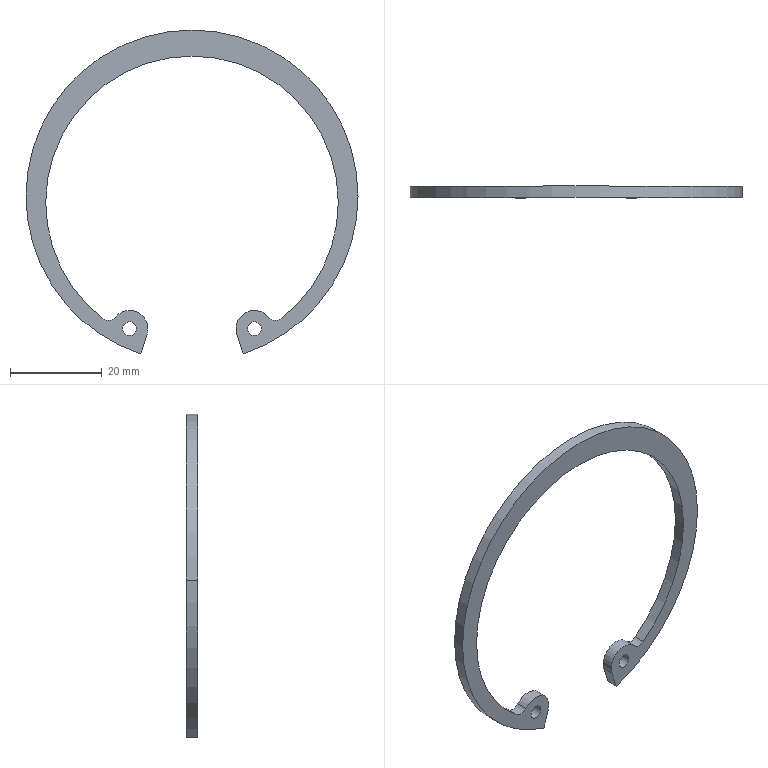Component | SolidWorks | BearingHousingAssembly-1_68HoleRetainingRing-1 | 1 solid | 19 faces | box 72.5 x 2.5 x 70.73 mm | volume 2284 mm3 | cylinder 15 | plane 4 | commonest cylinder face diameters 3 x4 72.5 x3 63.9 x3 8 x3 4 x2
STEP:
#1=CARTESIAN_POINT('',(-0.09511,7.097,-0.2362));
#2=VERTEX_POINT('',#1);
#3=CARTESIAN_POINT('',(-2.949,7.097,-0.2362));
#4=VERTEX_POINT('',#3);
#5=CARTESIAN_POINT('',(-1.522,7.097,-0.2362));
#6=DIRECTION('',(-0.,-1.,-0.));
#7=DIRECTION('',(1.,0.,-0.));
#8=AXIS2_PLACEMENT_3D('',#5,#6,#7);
#9=CIRCLE('',#8,1.427);
#10=EDGE_CURVE('',#2,#4,#9,.T.);
#11=ORIENTED_EDGE('',*,*,#10,.T.);
#12=CARTESIAN_POINT('',(-2.949,6.999,-0.2362));
#13=VERTEX_POINT('',#12);
#14=CARTESIAN_POINT('',(-2.949,7.097,-0.2362));
#15=DIRECTION('',(-0.,-1.,-0.));
#16=VECTOR('',#15,39.37);
#17=LINE('',#14,#16);
#18=EDGE_CURVE('',#4,#13,#17,.T.);
#19=ORIENTED_EDGE('',*,*,#18,.T.);
#20=CARTESIAN_POINT('',(-0.09511,6.999,-0.2362));
#21=VERTEX_POINT('',#20);
#22=CARTESIAN_POINT('',(-1.522,6.999,-0.2362));
#23=DIRECTION('',(0.,1.,0.));
#24=DIRECTION('',(1.,0.,-0.));
#25=AXIS2_PLACEMENT_3D('',#22,#23,#24);
#26=CIRCLE('',#25,1.427);
#27=EDGE_CURVE('',#13,#21,#26,.T.);
#28=ORIENTED_EDGE('',*,*,#27,.T.);
#29=CARTESIAN_POINT('',(-0.09511,7.097,-0.2362));
#30=DIRECTION('',(-0.,-1.,-0.));
#31=VECTOR('',#30,39.37);
#32=LINE('',#29,#31);
#33=EDGE_CURVE('',#2,#21,#32,.T.);
#34=ORIENTED_EDGE('',*,*,#33,.F.);
#35=EDGE_LOOP('',(#11,#19,#28,#34));
#36=FACE_OUTER_BOUND('',#35,.T.);
#37=CARTESIAN_POINT('',(-1.522,7.097,-0.2362));
#38=DIRECTION('',(-0.,-1.,-0.));
#39=DIRECTION('',(1.,0.,-0.));
#40=AXIS2_PLACEMENT_3D('',#37,#38,#39);
#41=CYLINDRICAL_SURFACE('',#40,1.427);
#42=ADVANCED_FACE('',(#36),#41,.T.);
#43=CARTESIAN_POINT('',(-1.081,7.097,-1.594));
#44=VERTEX_POINT('',#43);
#45=CARTESIAN_POINT('',(-1.522,7.097,-0.2362));
#46=DIRECTION('',(-0.,-1.,-0.));
#47=DIRECTION('',(1.,0.,-0.));
#48=AXIS2_PLACEMENT_3D('',#45,#46,#47);
#49=CIRCLE('',#48,1.427);
#50=EDGE_CURVE('',#44,#2,#49,.T.);
#51=ORIENTED_EDGE('',*,*,#50,.T.);
#52=ORIENTED_EDGE('',*,*,#33,.T.);
#53=CARTESIAN_POINT('',(-1.081,6.999,-1.594));
#54=VERTEX_POINT('',#53);
#55=CARTESIAN_POINT('',(-1.522,6.999,-0.2362));
#56=DIRECTION('',(0.,1.,0.));
#57=DIRECTION('',(1.,0.,-0.));
#58=AXIS2_PLACEMENT_3D('',#55,#56,#57);
#59=CIRCLE('',#58,1.427);
#60=EDGE_CURVE('',#21,#54,#59,.T.);
#61=ORIENTED_EDGE('',*,*,#60,.T.);
#62=CARTESIAN_POINT('',(-1.081,7.097,-1.594));
#63=DIRECTION('',(0.,1.,0.));
#64=VECTOR('',#63,39.37);
#65=LINE('',#62,#64);
#66=EDGE_CURVE('',#54,#44,#65,.T.);
#67=ORIENTED_EDGE('',*,*,#66,.T.);
#68=EDGE_LOOP('',(#51,#52,#61,#67));
#69=FACE_OUTER_BOUND('',#68,.T.);
#70=CARTESIAN_POINT('',(-1.522,7.097,-0.2362));
#71=DIRECTION('',(-0.,-1.,-0.));
#72=DIRECTION('',(1.,0.,-0.));
#73=AXIS2_PLACEMENT_3D('',#70,#71,#72);
#74=CYLINDRICAL_SURFACE('',#73,1.427);
#75=ADVANCED_FACE('',(#69),#74,.T.);
#76=CARTESIAN_POINT('',(-2.289,7.097,-1.289));
#77=VERTEX_POINT('',#76);
#78=CARTESIAN_POINT('',(-2.78,7.097,-0.2913));
#79=VERTEX_POINT('',#78);
#80=CARTESIAN_POINT('',(-1.522,7.097,-0.2913));
#81=DIRECTION('',(0.,1.,0.));
#82=DIRECTION('',(1.,0.,-0.));
#83=AXIS2_PLACEMENT_3D('',#80,#81,#82);
#84=CIRCLE('',#83,1.258);
#85=EDGE_CURVE('',#77,#79,#84,.T.);
#86=ORIENTED_EDGE('',*,*,#85,.T.);
#87=CARTESIAN_POINT('',(-2.78,6.999,-0.2913));
#88=VERTEX_POINT('',#87);
#89=CARTESIAN_POINT('',(-2.78,7.097,-0.2913));
#90=DIRECTION('',(-0.,-1.,-0.));
#91=VECTOR('',#90,39.37);
#92=LINE('',#89,#91);
#93=EDGE_CURVE('',#79,#88,#92,.T.);
#94=ORIENTED_EDGE('',*,*,#93,.T.);
#95=CARTESIAN_POINT('',(-2.289,6.999,-1.289));
#96=VERTEX_POINT('',#95);
#97=CARTESIAN_POINT('',(-1.522,6.999,-0.2913));
#98=DIRECTION('',(0.,1.,0.));
#99=DIRECTION('',(1.,0.,-0.));
#100=AXIS2_PLACEMENT_3D('',#97,#98,#99);
#101=CIRCLE('',#100,1.258);
#102=EDGE_CURVE('',#96,#88,#101,.T.);
#103=ORIENTED_EDGE('',*,*,#102,.F.);
#104=CARTESIAN_POINT('',(-2.289,7.097,-1.289));
#105=DIRECTION('',(-0.,-1.,-0.));
#106=VECTOR('',#105,39.37);
#107=LINE('',#104,#106);
#108=EDGE_CURVE('',#77,#96,#107,.T.);
#109=ORIENTED_EDGE('',*,*,#108,.F.);
#110=EDGE_LOOP('',(#86,#94,#103,#109));
#111=FACE_OUTER_BOUND('',#110,.T.);
#112=CARTESIAN_POINT('',(-1.522,7.097,-0.2913));
#113=DIRECTION('',(-0.,-1.,-0.));
#114=DIRECTION('',(1.,0.,-0.));
#115=AXIS2_PLACEMENT_3D('',#112,#113,#114);
#116=CYLINDRICAL_SURFACE('',#115,1.258);
#117=ADVANCED_FACE('',(#111),#116,.F.);
#118=ORIENTED_EDGE('',*,*,#93,.F.);
#119=CARTESIAN_POINT('',(-0.2644,7.097,-0.2913));
#120=VERTEX_POINT('',#119);
#121=CARTESIAN_POINT('',(-1.522,7.097,-0.2913));
#122=DIRECTION('',(0.,1.,0.));
#123=DIRECTION('',(1.,0.,-0.));
#124=AXIS2_PLACEMENT_3D('',#121,#122,#123);
#125=CIRCLE('',#124,1.258);
#126=EDGE_CURVE('',#79,#120,#125,.T.);
#127=ORIENTED_EDGE('',*,*,#126,.T.);
#128=CARTESIAN_POINT('',(-0.2644,6.999,-0.2913));
#129=VERTEX_POINT('',#128);
#130=CARTESIAN_POINT('',(-0.2644,7.097,-0.2913));
#131=DIRECTION('',(-0.,-1.,-0.));
#132=VECTOR('',#131,39.37);
#133=LINE('',#130,#132);
#134=EDGE_CURVE('',#120,#129,#133,.T.);
#135=ORIENTED_EDGE('',*,*,#134,.T.);
#136=CARTESIAN_POINT('',(-1.522,6.999,-0.2913));
#137=DIRECTION('',(0.,1.,0.));
#138=DIRECTION('',(1.,0.,-0.));
#139=AXIS2_PLACEMENT_3D('',#136,#137,#138);
#140=CIRCLE('',#139,1.258);
#141=EDGE_CURVE('',#88,#129,#140,.T.);
#142=ORIENTED_EDGE('',*,*,#141,.F.);
#143=EDGE_LOOP('',(#118,#127,#135,#142));
#144=FACE_OUTER_BOUND('',#143,.T.);
#145=CARTESIAN_POINT('',(-1.522,7.097,-0.2913));
#146=DIRECTION('',(-0.,-1.,-0.));
#147=DIRECTION('',(1.,0.,-0.));
#148=AXIS2_PLACEMENT_3D('',#145,#146,#147);
#149=CYLINDRICAL_SURFACE('',#148,1.258);
#150=ADVANCED_FACE('',(#144),#149,.F.);
#151=CARTESIAN_POINT('',(-1.909,7.097,-1.425));
#152=VERTEX_POINT('',#151);
#153=CARTESIAN_POINT('',(-1.901,7.097,-1.376));
#154=VERTEX_POINT('',#153);
#155=CARTESIAN_POINT('',(-2.058,7.097,-1.376));
#156=DIRECTION('',(-0.,-1.,-0.));
#157=DIRECTION('',(1.,0.,-0.));
#158=AXIS2_PLACEMENT_3D('',#155,#156,#157);
#159=CIRCLE('',#158,0.1575);
#160=EDGE_CURVE('',#152,#154,#159,.T.);
#161=ORIENTED_EDGE('',*,*,#160,.T.);
#162=CARTESIAN_POINT('',(-1.901,6.999,-1.376));
#163=VERTEX_POINT('',#162);
#164=CARTESIAN_POINT('',(-1.901,7.097,-1.376));
#165=DIRECTION('',(-0.,-1.,-0.));
#166=VECTOR('',#165,39.37);
#167=LINE('',#164,#166);
#168=EDGE_CURVE('',#154,#163,#167,.T.);
#169=ORIENTED_EDGE('',*,*,#168,.T.);
#170=CARTESIAN_POINT('',(-1.909,6.999,-1.425));
#171=VERTEX_POINT('',#170);
#172=CARTESIAN_POINT('',(-2.058,6.999,-1.376));
#173=DIRECTION('',(0.,1.,0.));
#174=DIRECTION('',(1.,0.,-0.));
#175=AXIS2_PLACEMENT_3D('',#172,#173,#174);
#176=CIRCLE('',#175,0.1575);
#177=EDGE_CURVE('',#163,#171,#176,.T.);
#178=ORIENTED_EDGE('',*,*,#177,.T.);
#179=CARTESIAN_POINT('',(-1.909,7.097,-1.425));
#180=DIRECTION('',(-0.,-1.,-0.));
#181=VECTOR('',#180,39.37);
#182=LINE('',#179,#181);
#183=EDGE_CURVE('',#152,#171,#182,.T.);
#184=ORIENTED_EDGE('',*,*,#183,.F.);
#185=EDGE_LOOP('',(#161,#169,#178,#184));
#186=FACE_OUTER_BOUND('',#185,.T.);
#187=CARTESIAN_POINT('',(-2.058,7.097,-1.376));
#188=DIRECTION('',(-0.,-1.,-0.));
#189=DIRECTION('',(1.,0.,-0.));
#190=AXIS2_PLACEMENT_3D('',#187,#188,#189);
#191=CYLINDRICAL_SURFACE('',#190,0.1575);
#192=ADVANCED_FACE('',(#186),#191,.T.);
#193=CARTESIAN_POINT('',(-0.9272,7.097,-1.376));
#194=VERTEX_POINT('',#193);
#195=CARTESIAN_POINT('',(-1.045,7.097,-1.376));
#196=VERTEX_POINT('',#195);
#197=CARTESIAN_POINT('',(-0.9862,7.097,-1.376));
#198=DIRECTION('',(0.,1.,0.));
#199=DIRECTION('',(1.,0.,-0.));
#200=AXIS2_PLACEMENT_3D('',#197,#198,#199);
#201=CIRCLE('',#200,0.05906);
#202=EDGE_CURVE('',#194,#196,#201,.T.);
#203=ORIENTED_EDGE('',*,*,#202,.T.);
#204=CARTESIAN_POINT('',(-1.045,6.999,-1.376));
#205=VERTEX_POINT('',#204);
#206=CARTESIAN_POINT('',(-1.045,7.097,-1.376));
#207=DIRECTION('',(-0.,-1.,-0.));
#208=VECTOR('',#207,39.37);
#209=LINE('',#206,#208);
#210=EDGE_CURVE('',#196,#205,#209,.T.);
#211=ORIENTED_EDGE('',*,*,#210,.T.);
#212=CARTESIAN_POINT('',(-0.9272,6.999,-1.376));
#213=VERTEX_POINT('',#212);
#214=CARTESIAN_POINT('',(-0.9862,6.999,-1.376));
#215=DIRECTION('',(0.,1.,0.));
#216=DIRECTION('',(1.,0.,-0.));
#217=AXIS2_PLACEMENT_3D('',#214,#215,#216);
#218=CIRCLE('',#217,0.05906);
#219=EDGE_CURVE('',#213,#205,#218,.T.);
#220=ORIENTED_EDGE('',*,*,#219,.F.);
#221=CARTESIAN_POINT('',(-0.9272,7.097,-1.376));
#222=DIRECTION('',(-0.,-1.,-0.));
#223=VECTOR('',#222,39.37);
#224=LINE('',#221,#223);
#225=EDGE_CURVE('',#194,#213,#224,.T.);
#226=ORIENTED_EDGE('',*,*,#225,.F.);
#227=EDGE_LOOP('',(#203,#211,#220,#226));
#228=FACE_OUTER_BOUND('',#227,.T.);
#229=CARTESIAN_POINT('',(-0.9862,7.097,-1.376));
#230=DIRECTION('',(-0.,-1.,-0.));
#231=DIRECTION('',(1.,0.,-0.));
#232=AXIS2_PLACEMENT_3D('',#229,#230,#231);
#233=CYLINDRICAL_SURFACE('',#232,0.05906);
#234=ADVANCED_FACE('',(#228),#233,.F.);
#235=CARTESIAN_POINT('',(-1.999,7.097,-1.376));
#236=VERTEX_POINT('',#235);
#237=CARTESIAN_POINT('',(-2.117,7.097,-1.376));
#238=VERTEX_POINT('',#237);
#239=CARTESIAN_POINT('',(-2.058,7.097,-1.376));
#240=DIRECTION('',(0.,1.,0.));
#241=DIRECTION('',(1.,0.,-0.));
#242=AXIS2_PLACEMENT_3D('',#239,#240,#241);
#243=CIRCLE('',#242,0.05906);
#244=EDGE_CURVE('',#236,#238,#243,.T.);
#245=ORIENTED_EDGE('',*,*,#244,.T.);
#246=CARTESIAN_POINT('',(-2.117,6.999,-1.376));
#247=VERTEX_POINT('',#246);
#248=CARTESIAN_POINT('',(-2.117,7.097,-1.376));
#249=DIRECTION('',(-0.,-1.,-0.));
#250=VECTOR('',#249,39.37);
#251=LINE('',#248,#250);
#252=EDGE_CURVE('',#238,#247,#251,.T.);
#253=ORIENTED_EDGE('',*,*,#252,.T.);
#254=CARTESIAN_POINT('',(-1.999,6.999,-1.376));
#255=VERTEX_POINT('',#254);
#256=CARTESIAN_POINT('',(-2.058,6.999,-1.376));
#257=DIRECTION('',(0.,1.,0.));
#258=DIRECTION('',(1.,0.,-0.));
#259=AXIS2_PLACEMENT_3D('',#256,#257,#258);
#260=CIRCLE('',#259,0.05906);
#261=EDGE_CURVE('',#255,#247,#260,.T.);
#262=ORIENTED_EDGE('',*,*,#261,.F.);
#263=CARTESIAN_POINT('',(-1.999,7.097,-1.376));
#264=DIRECTION('',(-0.,-1.,-0.));
#265=VECTOR('',#264,39.37);
#266=LINE('',#263,#265);
#267=EDGE_CURVE('',#236,#255,#266,.T.);
#268=ORIENTED_EDGE('',*,*,#267,.F.);
#269=EDGE_LOOP('',(#245,#253,#262,#268));
#270=FACE_OUTER_BOUND('',#269,.T.);
#271=CARTESIAN_POINT('',(-2.058,7.097,-1.376));
#272=DIRECTION('',(-0.,-1.,-0.));
#273=DIRECTION('',(1.,0.,-0.));
#274=AXIS2_PLACEMENT_3D('',#271,#272,#273);
#275=CYLINDRICAL_SURFACE('',#274,0.05906);
#276=ADVANCED_FACE('',(#270),#275,.F.);
#277=CARTESIAN_POINT('',(-1.136,7.097,-1.425));
#278=VERTEX_POINT('',#277);
#279=CARTESIAN_POINT('',(-1.136,7.097,-1.425));
#280=DIRECTION('',(0.309,-0.,-0.9511));
#281=VECTOR('',#280,39.37);
#282=LINE('',#279,#281);
#283=EDGE_CURVE('',#278,#44,#282,.T.);
#284=ORIENTED_EDGE('',*,*,#283,.F.);
#285=CARTESIAN_POINT('',(-0.8646,7.097,-1.276));
#286=VERTEX_POINT('',#285);
#287=CARTESIAN_POINT('',(-0.9862,7.097,-1.376));
#288=DIRECTION('',(-0.,-1.,-0.));
#289=DIRECTION('',(1.,0.,-0.));
#290=AXIS2_PLACEMENT_3D('',#287,#288,#289);
#291=CIRCLE('',#290,0.1575);
#292=EDGE_CURVE('',#286,#278,#291,.T.);
#293=ORIENTED_EDGE('',*,*,#292,.F.);
#294=CARTESIAN_POINT('',(-0.7558,7.097,-1.289));
#295=VERTEX_POINT('',#294);
#296=CARTESIAN_POINT('',(-0.8038,7.097,-1.226));
#297=DIRECTION('',(0.,1.,0.));
#298=DIRECTION('',(1.,0.,-0.));
#299=AXIS2_PLACEMENT_3D('',#296,#297,#298);
#300=CIRCLE('',#299,0.07874);
#301=EDGE_CURVE('',#295,#286,#300,.T.);
#302=ORIENTED_EDGE('',*,*,#301,.F.);
#303=CARTESIAN_POINT('',(-1.522,7.097,-0.2913));
#304=DIRECTION('',(0.,1.,0.));
#305=DIRECTION('',(1.,0.,-0.));
#306=AXIS2_PLACEMENT_3D('',#303,#304,#305);
#307=CIRCLE('',#306,1.258);
#308=EDGE_CURVE('',#120,#295,#307,.T.);
#309=ORIENTED_EDGE('',*,*,#308,.F.);
#310=ORIENTED_EDGE('',*,*,#126,.F.);
#311=ORIENTED_EDGE('',*,*,#85,.F.);
#312=CARTESIAN_POINT('',(-2.18,7.097,-1.276));
#313=VERTEX_POINT('',#312);
#314=CARTESIAN_POINT('',(-2.241,7.097,-1.226));
#315=DIRECTION('',(0.,1.,0.));
#316=DIRECTION('',(1.,0.,-0.));
#317=AXIS2_PLACEMENT_3D('',#314,#315,#316);
#318=CIRCLE('',#317,0.07874);
#319=EDGE_CURVE('',#313,#77,#318,.T.);
#320=ORIENTED_EDGE('',*,*,#319,.F.);
#321=CARTESIAN_POINT('',(-2.058,7.097,-1.376));
#322=DIRECTION('',(-0.,-1.,-0.));
#323=DIRECTION('',(1.,0.,-0.));
#324=AXIS2_PLACEMENT_3D('',#321,#322,#323);
#325=CIRCLE('',#324,0.1575);
#326=EDGE_CURVE('',#154,#313,#325,.T.);
#327=ORIENTED_EDGE('',*,*,#326,.F.);
#328=ORIENTED_EDGE('',*,*,#160,.F.);
#329=CARTESIAN_POINT('',(-1.963,7.097,-1.594));
#330=VERTEX_POINT('',#329);
#331=CARTESIAN_POINT('',(-1.963,7.097,-1.594));
#332=DIRECTION('',(0.309,-0.,0.9511));
#333=VECTOR('',#332,39.37);
#334=LINE('',#331,#333);
#335=EDGE_CURVE('',#330,#152,#334,.T.);
#336=ORIENTED_EDGE('',*,*,#335,.F.);
#337=CARTESIAN_POINT('',(-1.522,7.097,-0.2362));
#338=DIRECTION('',(-0.,-1.,-0.));
#339=DIRECTION('',(1.,0.,-0.));
#340=AXIS2_PLACEMENT_3D('',#337,#338,#339);
#341=CIRCLE('',#340,1.427);
#342=EDGE_CURVE('',#4,#330,#341,.T.);
#343=ORIENTED_EDGE('',*,*,#342,.F.);
#344=ORIENTED_EDGE('',*,*,#10,.F.);
#345=ORIENTED_EDGE('',*,*,#50,.F.);
#346=EDGE_LOOP('',(#284,#293,#302,#309,#310,#311,#320,#327,#328,#336,#343,#344,#345));
#347=FACE_OUTER_BOUND('',#346,.T.);
#348=ORIENTED_EDGE('',*,*,#202,.F.);
#349=CARTESIAN_POINT('',(-0.9862,7.097,-1.376));
#350=DIRECTION('',(0.,1.,0.));
#351=DIRECTION('',(1.,0.,-0.));
#352=AXIS2_PLACEMENT_3D('',#349,#350,#351);
#353=CIRCLE('',#352,0.05906);
#354=EDGE_CURVE('',#196,#194,#353,.T.);
#355=ORIENTED_EDGE('',*,*,#354,.F.);
#356=EDGE_LOOP('',(#348,#355));
#357=FACE_BOUND('',#356,.T.);
#358=ORIENTED_EDGE('',*,*,#244,.F.);
#359=CARTESIAN_POINT('',(-2.058,7.097,-1.376));
#360=DIRECTION('',(0.,1.,0.));
#361=DIRECTION('',(1.,0.,-0.));
#362=AXIS2_PLACEMENT_3D('',#359,#360,#361);
#363=CIRCLE('',#362,0.05906);
#364=EDGE_CURVE('',#238,#236,#363,.T.);
#365=ORIENTED_EDGE('',*,*,#364,.F.);
#366=EDGE_LOOP('',(#358,#365));
#367=FACE_BOUND('',#366,.T.);
#368=CARTESIAN_POINT('',(-1.522,7.097,-0.2362));
#369=DIRECTION('',(-0.,-1.,-0.));
#370=DIRECTION('',(1.,-0.,-0.));
#371=AXIS2_PLACEMENT_3D('',#368,#369,#370);
#372=PLANE('',#371);
#373=ADVANCED_FACE('',(#347,#357,#367),#372,.F.);
#374=ORIENTED_EDGE('',*,*,#18,.F.);
#375=ORIENTED_EDGE('',*,*,#342,.T.);
#376=CARTESIAN_POINT('',(-1.963,6.999,-1.594));
#377=VERTEX_POINT('',#376);
#378=CARTESIAN_POINT('',(-1.963,7.097,-1.594));
#379=DIRECTION('',(0.,1.,0.));
#380=VECTOR('',#379,39.37);
#381=LINE('',#378,#380);
#382=EDGE_CURVE('',#377,#330,#381,.T.);
#383=ORIENTED_EDGE('',*,*,#382,.F.);
#384=CARTESIAN_POINT('',(-1.522,6.999,-0.2362));
#385=DIRECTION('',(0.,1.,0.));
#386=DIRECTION('',(1.,0.,-0.));
#387=AXIS2_PLACEMENT_3D('',#384,#385,#386);
#388=CIRCLE('',#387,1.427);
#389=EDGE_CURVE('',#377,#13,#388,.T.);
#390=ORIENTED_EDGE('',*,*,#389,.T.);
#391=EDGE_LOOP('',(#374,#375,#383,#390));
#392=FACE_OUTER_BOUND('',#391,.T.);
#393=CARTESIAN_POINT('',(-1.522,7.097,-0.2362));
#394=DIRECTION('',(-0.,-1.,-0.));
#395=DIRECTION('',(1.,0.,-0.));
#396=AXIS2_PLACEMENT_3D('',#393,#394,#395);
#397=CYLINDRICAL_SURFACE('',#396,1.427);
#398=ADVANCED_FACE('',(#392),#397,.T.);
#399=ORIENTED_EDGE('',*,*,#283,.T.);
#400=ORIENTED_EDGE('',*,*,#66,.F.);
#401=CARTESIAN_POINT('',(-1.136,6.999,-1.425));
#402=VERTEX_POINT('',#401);
#403=CARTESIAN_POINT('',(-1.136,6.999,-1.425));
#404=DIRECTION('',(-0.309,0.,0.9511));
#405=VECTOR('',#404,39.37);
#406=LINE('',#403,#405);
#407=EDGE_CURVE('',#54,#402,#406,.T.);
#408=ORIENTED_EDGE('',*,*,#407,.T.);
#409=CARTESIAN_POINT('',(-1.136,7.097,-1.425));
#410=DIRECTION('',(0.,1.,0.));
#411=VECTOR('',#410,39.37);
#412=LINE('',#409,#411);
#413=EDGE_CURVE('',#402,#278,#412,.T.);
#414=ORIENTED_EDGE('',*,*,#413,.T.);
#415=EDGE_LOOP('',(#399,#400,#408,#414));
#416=FACE_OUTER_BOUND('',#415,.T.);
#417=CARTESIAN_POINT('',(-1.136,7.097,-1.425));
#418=DIRECTION('',(-0.9511,0.,-0.309));
#419=DIRECTION('',(0.309,-0.,-0.9511));
#420=AXIS2_PLACEMENT_3D('',#417,#418,#419);
#421=PLANE('',#420);
#422=ADVANCED_FACE('',(#416),#421,.T.);
#423=ORIENTED_EDGE('',*,*,#292,.T.);
#424=ORIENTED_EDGE('',*,*,#413,.F.);
#425=CARTESIAN_POINT('',(-0.8646,6.999,-1.276));
#426=VERTEX_POINT('',#425);
#427=CARTESIAN_POINT('',(-0.9862,6.999,-1.376));
#428=DIRECTION('',(0.,1.,0.));
#429=DIRECTION('',(1.,0.,-0.));
#430=AXIS2_PLACEMENT_3D('',#427,#428,#429);
#431=CIRCLE('',#430,0.1575);
#432=EDGE_CURVE('',#402,#426,#431,.T.);
#433=ORIENTED_EDGE('',*,*,#432,.T.);
#434=CARTESIAN_POINT('',(-0.8646,7.097,-1.276));
#435=DIRECTION('',(0.,1.,0.));
#436=VECTOR('',#435,39.37);
#437=LINE('',#434,#436);
#438=EDGE_CURVE('',#426,#286,#437,.T.);
#439=ORIENTED_EDGE('',*,*,#438,.T.);
#440=EDGE_LOOP('',(#423,#424,#433,#439));
#441=FACE_OUTER_BOUND('',#440,.T.);
#442=CARTESIAN_POINT('',(-0.9862,7.097,-1.376));
#443=DIRECTION('',(-0.,-1.,-0.));
#444=DIRECTION('',(1.,0.,-0.));
#445=AXIS2_PLACEMENT_3D('',#442,#443,#444);
#446=CYLINDRICAL_SURFACE('',#445,0.1575);
#447=ADVANCED_FACE('',(#441),#446,.T.);
#448=CARTESIAN_POINT('',(-0.7558,6.999,-1.289));
#449=VERTEX_POINT('',#448);
#450=CARTESIAN_POINT('',(-0.7558,7.097,-1.289));
#451=DIRECTION('',(-0.,-1.,-0.));
#452=VECTOR('',#451,39.37);
#453=LINE('',#450,#452);
#454=EDGE_CURVE('',#295,#449,#453,.T.);
#455=ORIENTED_EDGE('',*,*,#454,.F.);
#456=ORIENTED_EDGE('',*,*,#301,.T.);
#457=ORIENTED_EDGE('',*,*,#438,.F.);
#458=CARTESIAN_POINT('',(-0.8038,6.999,-1.226));
#459=DIRECTION('',(0.,1.,0.));
#460=DIRECTION('',(1.,0.,-0.));
#461=AXIS2_PLACEMENT_3D('',#458,#459,#460);
#462=CIRCLE('',#461,0.07874);
#463=EDGE_CURVE('',#449,#426,#462,.T.);
#464=ORIENTED_EDGE('',*,*,#463,.F.);
#465=EDGE_LOOP('',(#455,#456,#457,#464));
#466=FACE_OUTER_BOUND('',#465,.T.);
#467=CARTESIAN_POINT('',(-0.8038,7.097,-1.226));
#468=DIRECTION('',(-0.,-1.,-0.));
#469=DIRECTION('',(1.,0.,-0.));
#470=AXIS2_PLACEMENT_3D('',#467,#468,#469);
#471=CYLINDRICAL_SURFACE('',#470,0.07874);
#472=ADVANCED_FACE('',(#466),#471,.F.);
#473=ORIENTED_EDGE('',*,*,#134,.F.);
#474=ORIENTED_EDGE('',*,*,#308,.T.);
#475=ORIENTED_EDGE('',*,*,#454,.T.);
#476=CARTESIAN_POINT('',(-1.522,6.999,-0.2913));
#477=DIRECTION('',(0.,1.,0.));
#478=DIRECTION('',(1.,0.,-0.));
#479=AXIS2_PLACEMENT_3D('',#476,#477,#478);
#480=CIRCLE('',#479,1.258);
#481=EDGE_CURVE('',#129,#449,#480,.T.);
#482=ORIENTED_EDGE('',*,*,#481,.F.);
#483=EDGE_LOOP('',(#473,#474,#475,#482));
#484=FACE_OUTER_BOUND('',#483,.T.);
#485=CARTESIAN_POINT('',(-1.522,7.097,-0.2913));
#486=DIRECTION('',(-0.,-1.,-0.));
#487=DIRECTION('',(1.,0.,-0.));
#488=AXIS2_PLACEMENT_3D('',#485,#486,#487);
#489=CYLINDRICAL_SURFACE('',#488,1.258);
#490=ADVANCED_FACE('',(#484),#489,.F.);
#491=CARTESIAN_POINT('',(-2.18,6.999,-1.276));
#492=VERTEX_POINT('',#491);
#493=CARTESIAN_POINT('',(-2.18,7.097,-1.276));
#494=DIRECTION('',(-0.,-1.,-0.));
#495=VECTOR('',#494,39.37);
#496=LINE('',#493,#495);
#497=EDGE_CURVE('',#313,#492,#496,.T.);
#498=ORIENTED_EDGE('',*,*,#497,.F.);
#499=ORIENTED_EDGE('',*,*,#319,.T.);
#500=ORIENTED_EDGE('',*,*,#108,.T.);
#501=CARTESIAN_POINT('',(-2.241,6.999,-1.226));
#502=DIRECTION('',(0.,1.,0.));
#503=DIRECTION('',(1.,0.,-0.));
#504=AXIS2_PLACEMENT_3D('',#501,#502,#503);
#505=CIRCLE('',#504,0.07874);
#506=EDGE_CURVE('',#492,#96,#505,.T.);
#507=ORIENTED_EDGE('',*,*,#506,.F.);
#508=EDGE_LOOP('',(#498,#499,#500,#507));
#509=FACE_OUTER_BOUND('',#508,.T.);
#510=CARTESIAN_POINT('',(-2.241,7.097,-1.226));
#511=DIRECTION('',(-0.,-1.,-0.));
#512=DIRECTION('',(1.,0.,-0.));
#513=AXIS2_PLACEMENT_3D('',#510,#511,#512);
#514=CYLINDRICAL_SURFACE('',#513,0.07874);
#515=ADVANCED_FACE('',(#509),#514,.F.);
#516=ORIENTED_EDGE('',*,*,#168,.F.);
#517=ORIENTED_EDGE('',*,*,#326,.T.);
#518=ORIENTED_EDGE('',*,*,#497,.T.);
#519=CARTESIAN_POINT('',(-2.058,6.999,-1.376));
#520=DIRECTION('',(0.,1.,0.));
#521=DIRECTION('',(1.,0.,-0.));
#522=AXIS2_PLACEMENT_3D('',#519,#520,#521);
#523=CIRCLE('',#522,0.1575);
#524=EDGE_CURVE('',#492,#163,#523,.T.);
#525=ORIENTED_EDGE('',*,*,#524,.T.);
#526=EDGE_LOOP('',(#516,#517,#518,#525));
#527=FACE_OUTER_BOUND('',#526,.T.);
#528=CARTESIAN_POINT('',(-2.058,7.097,-1.376));
#529=DIRECTION('',(-0.,-1.,-0.));
#530=DIRECTION('',(1.,0.,-0.));
#531=AXIS2_PLACEMENT_3D('',#528,#529,#530);
#532=CYLINDRICAL_SURFACE('',#531,0.1575);
#533=ADVANCED_FACE('',(#527),#532,.T.);
#534=ORIENTED_EDGE('',*,*,#335,.T.);
#535=ORIENTED_EDGE('',*,*,#183,.T.);
#536=CARTESIAN_POINT('',(-1.909,6.999,-1.425));
#537=DIRECTION('',(-0.309,0.,-0.9511));
#538=VECTOR('',#537,39.37);
#539=LINE('',#536,#538);
#540=EDGE_CURVE('',#171,#377,#539,.T.);
#541=ORIENTED_EDGE('',*,*,#540,.T.);
#542=ORIENTED_EDGE('',*,*,#382,.T.);
#543=EDGE_LOOP('',(#534,#535,#541,#542));
#544=FACE_OUTER_BOUND('',#543,.T.);
#545=CARTESIAN_POINT('',(-1.909,7.097,-1.425));
#546=DIRECTION('',(0.9511,-0.,-0.309));
#547=DIRECTION('',(0.309,-0.,0.9511));
#548=AXIS2_PLACEMENT_3D('',#545,#546,#547);
#549=PLANE('',#548);
#550=ADVANCED_FACE('',(#544),#549,.T.);
#551=ORIENTED_EDGE('',*,*,#210,.F.);
#552=ORIENTED_EDGE('',*,*,#354,.T.);
#553=ORIENTED_EDGE('',*,*,#225,.T.);
#554=CARTESIAN_POINT('',(-0.9862,6.999,-1.376));
#555=DIRECTION('',(0.,1.,0.));
#556=DIRECTION('',(1.,0.,-0.));
#557=AXIS2_PLACEMENT_3D('',#554,#555,#556);
#558=CIRCLE('',#557,0.05906);
#559=EDGE_CURVE('',#205,#213,#558,.T.);
#560=ORIENTED_EDGE('',*,*,#559,.F.);
#561=EDGE_LOOP('',(#551,#552,#553,#560));
#562=FACE_OUTER_BOUND('',#561,.T.);
#563=CARTESIAN_POINT('',(-0.9862,7.097,-1.376));
#564=DIRECTION('',(-0.,-1.,-0.));
#565=DIRECTION('',(1.,0.,-0.));
#566=AXIS2_PLACEMENT_3D('',#563,#564,#565);
#567=CYLINDRICAL_SURFACE('',#566,0.05906);
#568=ADVANCED_FACE('',(#562),#567,.F.);
#569=ORIENTED_EDGE('',*,*,#252,.F.);
#570=ORIENTED_EDGE('',*,*,#364,.T.);
#571=ORIENTED_EDGE('',*,*,#267,.T.);
#572=CARTESIAN_POINT('',(-2.058,6.999,-1.376));
#573=DIRECTION('',(0.,1.,0.));
#574=DIRECTION('',(1.,0.,-0.));
#575=AXIS2_PLACEMENT_3D('',#572,#573,#574);
#576=CIRCLE('',#575,0.05906);
#577=EDGE_CURVE('',#247,#255,#576,.T.);
#578=ORIENTED_EDGE('',*,*,#577,.F.);
#579=EDGE_LOOP('',(#569,#570,#571,#578));
#580=FACE_OUTER_BOUND('',#579,.T.);
#581=CARTESIAN_POINT('',(-2.058,7.097,-1.376));
#582=DIRECTION('',(-0.,-1.,-0.));
#583=DIRECTION('',(1.,0.,-0.));
#584=AXIS2_PLACEMENT_3D('',#581,#582,#583);
#585=CYLINDRICAL_SURFACE('',#584,0.05906);
#586=ADVANCED_FACE('',(#580),#585,.F.);
#587=ORIENTED_EDGE('',*,*,#432,.F.);
#588=ORIENTED_EDGE('',*,*,#407,.F.);
#589=ORIENTED_EDGE('',*,*,#60,.F.);
#590=ORIENTED_EDGE('',*,*,#27,.F.);
#591=ORIENTED_EDGE('',*,*,#389,.F.);
#592=ORIENTED_EDGE('',*,*,#540,.F.);
#593=ORIENTED_EDGE('',*,*,#177,.F.);
#594=ORIENTED_EDGE('',*,*,#524,.F.);
#595=ORIENTED_EDGE('',*,*,#506,.T.);
#596=ORIENTED_EDGE('',*,*,#102,.T.);
#597=ORIENTED_EDGE('',*,*,#141,.T.);
#598=ORIENTED_EDGE('',*,*,#481,.T.);
#599=ORIENTED_EDGE('',*,*,#463,.T.);
#600=EDGE_LOOP('',(#587,#588,#589,#590,#591,#592,#593,#594,#595,#596,#597,#598,#599));
#601=FACE_OUTER_BOUND('',#600,.T.);
#602=ORIENTED_EDGE('',*,*,#219,.T.);
#603=ORIENTED_EDGE('',*,*,#559,.T.);
#604=EDGE_LOOP('',(#602,#603));
#605=FACE_BOUND('',#604,.T.);
#606=ORIENTED_EDGE('',*,*,#261,.T.);
#607=ORIENTED_EDGE('',*,*,#577,.T.);
#608=EDGE_LOOP('',(#606,#607));
#609=FACE_BOUND('',#608,.T.);
#610=CARTESIAN_POINT('',(-1.522,6.999,-0.2362));
#611=DIRECTION('',(-0.,-1.,-0.));
#612=DIRECTION('',(1.,-0.,-0.));
#613=AXIS2_PLACEMENT_3D('',#610,#611,#612);
#614=PLANE('',#613);
#615=ADVANCED_FACE('',(#601,#605,#609),#614,.T.);
#616=CLOSED_SHELL('',(#42,#75,#117,#150,#192,#234,#276,#373,#398,#422,#447,#472,#490,#515,#533,#550,#568,#586,#615));
#617=MANIFOLD_SOLID_BREP('',#616);
#618=CARTESIAN_POINT('',(0.,0.,0.));
#619=DIRECTION('',(0.,0.,1.));
#620=DIRECTION('',(1.,0.,0.));
#621=AXIS2_PLACEMENT_3D('',#618,#619,#620);
#622=(LENGTH_UNIT()NAMED_UNIT(*)SI_UNIT($,.METRE.));
#623=LENGTH_MEASURE_WITH_UNIT(LENGTH_MEASURE(0.0254),#622);
#624=DIMENSIONAL_EXPONENTS(1.,0.,0.,0.,0.,0.,0.);
#625=(CONVERSION_BASED_UNIT('',#623)LENGTH_UNIT()NAMED_UNIT(#624));
#626=UNCERTAINTY_MEASURE_WITH_UNIT(LENGTH_MEASURE(0.00001),#625,'','');
#627=(NAMED_UNIT(*)PLANE_ANGLE_UNIT()SI_UNIT($,.RADIAN.));
#628=(NAMED_UNIT(*)SI_UNIT($,.STERADIAN.)SOLID_ANGLE_UNIT());
#629=(GEOMETRIC_REPRESENTATION_CONTEXT(3)GLOBAL_UNCERTAINTY_ASSIGNED_CONTEXT((#626))GLOBAL_UNIT_ASSIGNED_CONTEXT((#625,#627,#628))REPRESENTATION_CONTEXT('',''));
#630=ADVANCED_BREP_SHAPE_REPRESENTATION('',(#617,#621),#629);
#631=COLOUR_RGB('',0.7922,0.8196,0.9333);
#632=FILL_AREA_STYLE_COLOUR('',#631);
#633=FILL_AREA_STYLE('',(#632));
#634=SURFACE_STYLE_FILL_AREA(#633);
#635=SURFACE_SIDE_STYLE('',(#634));
#636=SURFACE_STYLE_USAGE(.BOTH.,#635);
#637=PRESENTATION_STYLE_ASSIGNMENT((#636));
#638=STYLED_ITEM('',(#637),#617);
#639=(LENGTH_UNIT()NAMED_UNIT(*)SI_UNIT($,.METRE.));
#640=LENGTH_MEASURE_WITH_UNIT(LENGTH_MEASURE(0.0254),#639);
#641=DIMENSIONAL_EXPONENTS(1.,0.,0.,0.,0.,0.,0.);
#642=(CONVERSION_BASED_UNIT('',#640)LENGTH_UNIT()NAMED_UNIT(#641));
#643=UNCERTAINTY_MEASURE_WITH_UNIT(LENGTH_MEASURE(0.00001),#642,'','');
#644=(NAMED_UNIT(*)PLANE_ANGLE_UNIT()SI_UNIT($,.RADIAN.));
#645=(NAMED_UNIT(*)SI_UNIT($,.STERADIAN.)SOLID_ANGLE_UNIT());
#646=(GEOMETRIC_REPRESENTATION_CONTEXT(3)GLOBAL_UNCERTAINTY_ASSIGNED_CONTEXT((#643))GLOBAL_UNIT_ASSIGNED_CONTEXT((#642,#644,#645))REPRESENTATION_CONTEXT('',''));
#647=MECHANICAL_DESIGN_GEOMETRIC_PRESENTATION_REPRESENTATION('',(#638),#646);
#648=PRESENTATION_LAYER_ASSIGNMENT('','',(#638));